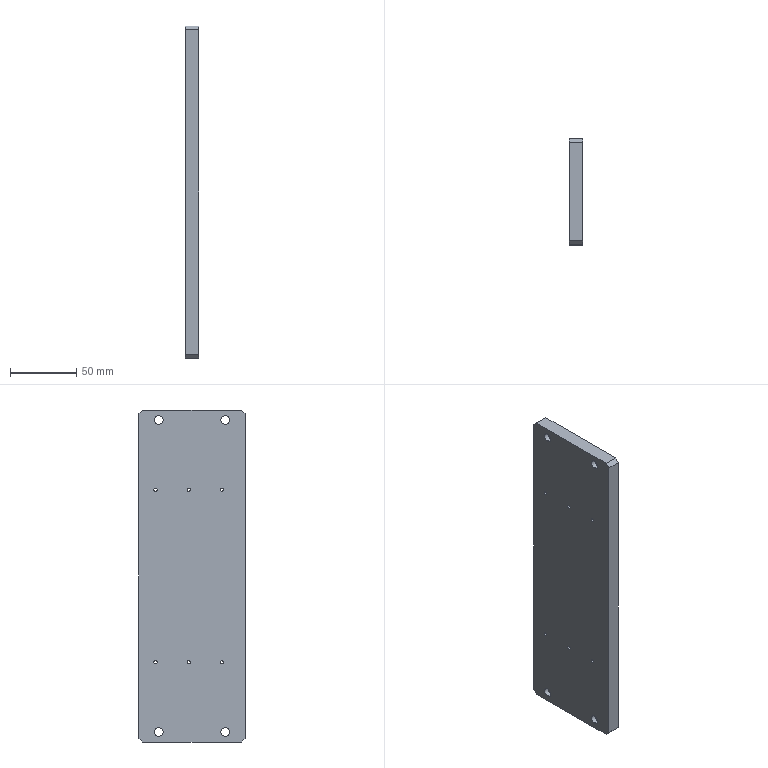Component | SolidWorks | 8TC-A15004-D0-10A-1 | 1 solid | 42 faces | box 10 x 80 x 250 mm | volume 196600 mm3 | cylinder 28 | plane 14 | commonest cylinder face diameters 2.5 x12 11 x8 6.6 x8 | material #45
build123d program:
from build123d import *

# Parameters (mm, degrees)
SKETCH1_W                                       = 80
SKETCH1_H                                       = 250
BOSS_EXTRUDE1_DEPTH                             = 5
CHAMFER1_SIZE                                   = 3
M3_TAPPED_HOLE1_D                               = 2.5
M6_HEX_SOCKET_HEAD_CAP_SCREW_CBORE1_D           = 6.6
M6_HEX_SOCKET_HEAD_CAP_SCREW_CBORE1_CBORE_D     = 11
M6_HEX_SOCKET_HEAD_CAP_SCREW_CBORE1_CBORE_DEPTH = 6.4


with BuildPart() as part:
    # Sketch1 → Boss-Extrude1 (new, symmetric)
    with BuildSketch(Plane(origin=(0, 0, 0), x_dir=(1, 0, 0), z_dir=(0, 1, 0))):
        Rectangle(SKETCH1_W, SKETCH1_H)
    extrude(amount=BOSS_EXTRUDE1_DEPTH, both=True)

    # Chamfer1
    chamfer1_edges = [part.edges().sort_by_distance(p)[0] for p in [
        (40, 0, 125),
        (-40, 0, 125),
        (-40, 0, -125),
        (40, 0, -125),
    ]]
    chamfer(chamfer1_edges, length=CHAMFER1_SIZE)

    # M3 Tapped Hole1 (through all)
    with Locations(Plane(origin=(0, 5, 0), x_dir=(1, 0, 0), z_dir=(0, 1, 0))):
        with Locations((22.5, 65), (-2.5, 65), (-27.5, 65), (22.5, -65), (-2.5, -65), (-27.5, -65)):
            Hole(M3_TAPPED_HOLE1_D / 2)

    # M6 Hex Socket Head Cap Screw CBORE1 (through all)
    with Locations(Plane(origin=(0, -5, 0), x_dir=(-1, 0, 0), z_dir=(0, -1, 0))):
        with Locations((-25, 117.5), (25, 117.5), (25, -117.5), (-25, -117.5)):
            CounterBoreHole(M6_HEX_SOCKET_HEAD_CAP_SCREW_CBORE1_D / 2, M6_HEX_SOCKET_HEAD_CAP_SCREW_CBORE1_CBORE_D / 2, M6_HEX_SOCKET_HEAD_CAP_SCREW_CBORE1_CBORE_DEPTH)


solid = part.part

# Placed as in the assembly
solid = solid.moved(Location((52.5, 380.5, 0), (180, 0, 90)))